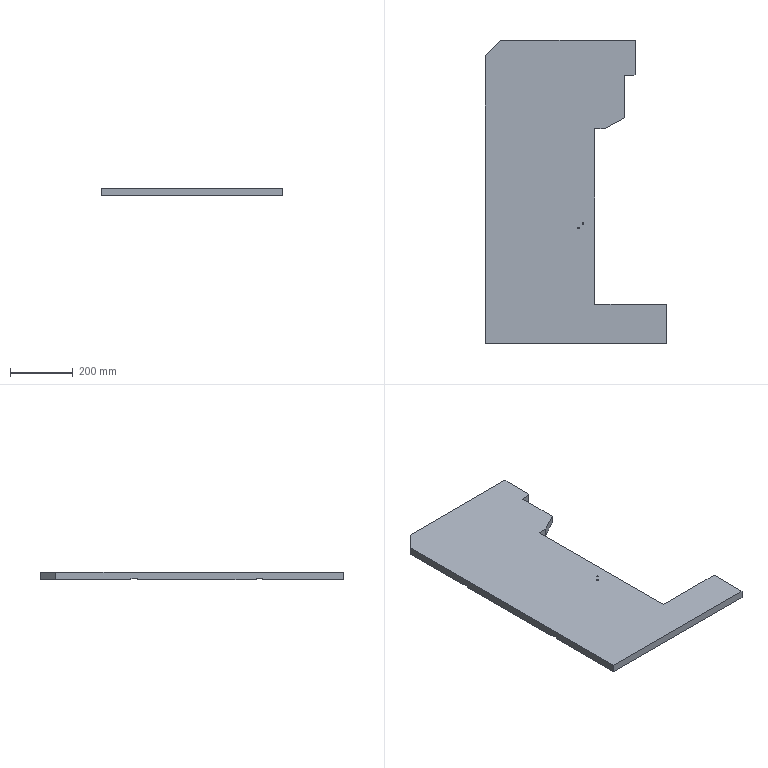Component | SolidWorks | 100-02-1 | 1 solid | 35 faces | box 580 x 970 x 25 mm | volume 9861709 mm3 | plane 23 | cylinder 8 | cone 4 | commonest cylinder face diameters 6.8 x4 5 x4 | material 45
build123d program:
from build123d import *

# Parameters (mm, degrees)
BOSS_EXTRUDE1_DEPTH   = 12.5
CHAMFER1_SIZE         = 5
M6_TAPPED_HOLE1_D     = 5
SKETCH6_W             = 350
SKETCH6_H             = 20
CUT_EXTRUDE1_DEPTH    = 4
LPATTERN1_COUNT       = 2
LPATTERN1_PITCH       = 400
M8_TAPPED_HOLE1_D     = 6.8
M8_TAPPED_HOLE1_DEPTH = 19.75
M8_TAPPED_HOLE1_TIP   = 2.043


with BuildPart() as part:
    # Sketch1 → Boss-Extrude1 (new, symmetric)
    with BuildSketch(Plane.XY):
        Polygon((580, 126), (350, 126), (350, 687), (380, 687), (445, 722), (445, 857), (479, 857), (479, 970), (50, 970), (0, 920), (0, 0), (580, 0), align=None)
    extrude(amount=BOSS_EXTRUDE1_DEPTH, both=True)

    # Chamfer1
    chamfer1_edges = [part.edges().sort_by_distance(p)[0] for p in [
        (479, 857, 0),
    ]]
    chamfer(chamfer1_edges, length=CHAMFER1_SIZE)

    # M6 Tapped Hole1 (through all)
    with Locations(Plane.XY.offset(12.5)):
        with Locations((298, 370), (312.142, 384.142)):
            Hole(M6_TAPPED_HOLE1_D / 2)

    # Sketch6 → Cut-Extrude1 (cut)
    with BuildSketch(Plane(origin=(0, 0, -12.5), x_dir=(-1, 0, 0), z_dir=(0, 0, -1))):
        with Locations((-175, 270)):
            Rectangle(SKETCH6_W, SKETCH6_H)
    cut_extrude1 = extrude(amount=-CUT_EXTRUDE1_DEPTH, mode=Mode.SUBTRACT)

    # LPattern1: Cut-Extrude1 ×2
    with Locations(*[(0, i * LPATTERN1_PITCH, 0) for i in range(1, LPATTERN1_COUNT)]):
        add(cut_extrude1, mode=Mode.SUBTRACT)

    # M8 Tapped Hole1
    with Locations(Plane(origin=(0, 126, 0), x_dir=(1, 0, 0), z_dir=(0, 1, 0))):
        with Locations((552.5, 0), (507.5, 0)):
            Hole(M8_TAPPED_HOLE1_D / 2, depth=M8_TAPPED_HOLE1_DEPTH)
            with Locations((0, 0, -(M8_TAPPED_HOLE1_DEPTH + M8_TAPPED_HOLE1_TIP / 2))):  # 118° drill point
                Cone(0, M8_TAPPED_HOLE1_D / 2, M8_TAPPED_HOLE1_TIP, mode=Mode.SUBTRACT)


solid = part.part

# Placed as in the assembly
solid = solid.moved(Location((-300, 14, 97.5), (0, 0, 0)))
STEP:
#1=COLOUR_RGB('',0.7922,0.8196,0.9333);
#2=FILL_AREA_STYLE_COLOUR('',#1);
#3=FILL_AREA_STYLE('',(#2));
#4=SURFACE_STYLE_FILL_AREA(#3);
#5=SURFACE_SIDE_STYLE('',(#4));
#6=SURFACE_STYLE_USAGE(.BOTH.,#5);
#7=PRESENTATION_STYLE_ASSIGNMENT((#6));
#8=CARTESIAN_POINT('',(9.941,4.734,3.705));
#9=VERTEX_POINT('',#8);
#10=CARTESIAN_POINT('',(9.941,4.734,3.972));
#11=VERTEX_POINT('',#10);
#12=CARTESIAN_POINT('',(9.941,4.734,3.839));
#13=DIRECTION('',(0.,1.,0.));
#14=DIRECTION('',(0.,0.,1.));
#15=AXIS2_PLACEMENT_3D('',#12,#13,#14);
#16=CIRCLE('',#15,0.1339);
#17=EDGE_CURVE('',#9,#11,#16,.T.);
#18=ORIENTED_EDGE('',*,*,#17,.F.);
#19=CARTESIAN_POINT('',(9.941,5.512,3.705));
#20=VERTEX_POINT('',#19);
#21=CARTESIAN_POINT('',(9.941,5.512,3.705));
#22=DIRECTION('',(0.,1.,0.));
#23=VECTOR('',#22,39.37);
#24=LINE('',#21,#23);
#25=EDGE_CURVE('',#9,#20,#24,.T.);
#26=ORIENTED_EDGE('',*,*,#25,.T.);
#27=CARTESIAN_POINT('',(9.941,5.512,3.972));
#28=VERTEX_POINT('',#27);
#29=CARTESIAN_POINT('',(9.941,5.512,3.839));
#30=DIRECTION('',(0.,1.,0.));
#31=DIRECTION('',(0.,0.,1.));
#32=AXIS2_PLACEMENT_3D('',#29,#30,#31);
#33=CIRCLE('',#32,0.1339);
#34=EDGE_CURVE('',#20,#28,#33,.T.);
#35=ORIENTED_EDGE('',*,*,#34,.T.);
#36=CARTESIAN_POINT('',(9.941,5.512,3.972));
#37=DIRECTION('',(0.,1.,0.));
#38=VECTOR('',#37,39.37);
#39=LINE('',#36,#38);
#40=EDGE_CURVE('',#11,#28,#39,.T.);
#41=ORIENTED_EDGE('',*,*,#40,.F.);
#42=EDGE_LOOP('',(#18,#26,#35,#41));
#43=FACE_OUTER_BOUND('',#42,.T.);
#44=CARTESIAN_POINT('',(9.941,5.512,3.839));
#45=DIRECTION('',(0.,1.,0.));
#46=DIRECTION('',(0.,0.,1.));
#47=AXIS2_PLACEMENT_3D('',#44,#45,#46);
#48=CYLINDRICAL_SURFACE('',#47,0.1339);
#49=ADVANCED_FACE('',(#43),#48,.F.);
#50=CARTESIAN_POINT('',(9.941,4.654,3.839));
#51=VERTEX_POINT('',#50);
#52=CARTESIAN_POINT('',(9.941,4.734,3.972));
#53=DIRECTION('',(0.,0.515,0.8572));
#54=VECTOR('',#53,39.37);
#55=LINE('',#52,#54);
#56=EDGE_CURVE('',#51,#11,#55,.T.);
#57=ORIENTED_EDGE('',*,*,#56,.F.);
#58=CARTESIAN_POINT('',(9.941,4.734,3.705));
#59=DIRECTION('',(0.,0.515,-0.8572));
#60=VECTOR('',#59,39.37);
#61=LINE('',#58,#60);
#62=EDGE_CURVE('',#51,#9,#61,.T.);
#63=ORIENTED_EDGE('',*,*,#62,.T.);
#64=ORIENTED_EDGE('',*,*,#17,.T.);
#65=EDGE_LOOP('',(#57,#63,#64));
#66=FACE_OUTER_BOUND('',#65,.T.);
#67=CARTESIAN_POINT('',(9.941,4.734,3.839));
#68=DIRECTION('',(0.,1.,0.));
#69=DIRECTION('',(0.,0.,1.));
#70=AXIS2_PLACEMENT_3D('',#67,#68,#69);
#71=CONICAL_SURFACE('',#70,0.1339,1.03);
#72=ADVANCED_FACE('',(#66),#71,.F.);
#73=CARTESIAN_POINT('',(8.169,4.734,3.705));
#74=VERTEX_POINT('',#73);
#75=CARTESIAN_POINT('',(8.169,4.734,3.972));
#76=VERTEX_POINT('',#75);
#77=CARTESIAN_POINT('',(8.169,4.734,3.839));
#78=DIRECTION('',(0.,1.,0.));
#79=DIRECTION('',(0.,0.,1.));
#80=AXIS2_PLACEMENT_3D('',#77,#78,#79);
#81=CIRCLE('',#80,0.1339);
#82=EDGE_CURVE('',#74,#76,#81,.T.);
#83=ORIENTED_EDGE('',*,*,#82,.F.);
#84=CARTESIAN_POINT('',(8.169,5.512,3.705));
#85=VERTEX_POINT('',#84);
#86=CARTESIAN_POINT('',(8.169,5.512,3.705));
#87=DIRECTION('',(0.,1.,0.));
#88=VECTOR('',#87,39.37);
#89=LINE('',#86,#88);
#90=EDGE_CURVE('',#74,#85,#89,.T.);
#91=ORIENTED_EDGE('',*,*,#90,.T.);
#92=CARTESIAN_POINT('',(8.169,5.512,3.972));
#93=VERTEX_POINT('',#92);
#94=CARTESIAN_POINT('',(8.169,5.512,3.839));
#95=DIRECTION('',(0.,1.,0.));
#96=DIRECTION('',(0.,0.,1.));
#97=AXIS2_PLACEMENT_3D('',#94,#95,#96);
#98=CIRCLE('',#97,0.1339);
#99=EDGE_CURVE('',#85,#93,#98,.T.);
#100=ORIENTED_EDGE('',*,*,#99,.T.);
#101=CARTESIAN_POINT('',(8.169,5.512,3.972));
#102=DIRECTION('',(0.,1.,0.));
#103=VECTOR('',#102,39.37);
#104=LINE('',#101,#103);
#105=EDGE_CURVE('',#76,#93,#104,.T.);
#106=ORIENTED_EDGE('',*,*,#105,.F.);
#107=EDGE_LOOP('',(#83,#91,#100,#106));
#108=FACE_OUTER_BOUND('',#107,.T.);
#109=CARTESIAN_POINT('',(8.169,5.512,3.839));
#110=DIRECTION('',(0.,1.,0.));
#111=DIRECTION('',(0.,0.,1.));
#112=AXIS2_PLACEMENT_3D('',#109,#110,#111);
#113=CYLINDRICAL_SURFACE('',#112,0.1339);
#114=ADVANCED_FACE('',(#108),#113,.F.);
#115=CARTESIAN_POINT('',(8.169,4.654,3.839));
#116=VERTEX_POINT('',#115);
#117=CARTESIAN_POINT('',(8.169,4.734,3.972));
#118=DIRECTION('',(0.,0.515,0.8572));
#119=VECTOR('',#118,39.37);
#120=LINE('',#117,#119);
#121=EDGE_CURVE('',#116,#76,#120,.T.);
#122=ORIENTED_EDGE('',*,*,#121,.F.);
#123=CARTESIAN_POINT('',(8.169,4.734,3.705));
#124=DIRECTION('',(0.,0.515,-0.8572));
#125=VECTOR('',#124,39.37);
#126=LINE('',#123,#125);
#127=EDGE_CURVE('',#116,#74,#126,.T.);
#128=ORIENTED_EDGE('',*,*,#127,.T.);
#129=ORIENTED_EDGE('',*,*,#82,.T.);
#130=EDGE_LOOP('',(#122,#128,#129));
#131=FACE_OUTER_BOUND('',#130,.T.);
#132=CARTESIAN_POINT('',(8.169,4.734,3.839));
#133=DIRECTION('',(0.,1.,0.));
#134=DIRECTION('',(0.,0.,1.));
#135=AXIS2_PLACEMENT_3D('',#132,#133,#134);
#136=CONICAL_SURFACE('',#135,0.1339,1.03);
#137=ADVANCED_FACE('',(#131),#136,.F.);
#138=CARTESIAN_POINT('',(-0.1772,15.118,3.346));
#139=VERTEX_POINT('',#138);
#140=CARTESIAN_POINT('',(0.01969,15.118,3.346));
#141=VERTEX_POINT('',#140);
#142=CARTESIAN_POINT('',(-0.07874,15.118,3.346));
#143=DIRECTION('',(0.,0.,1.));
#144=DIRECTION('',(1.,0.,0.));
#145=AXIS2_PLACEMENT_3D('',#142,#143,#144);
#146=CIRCLE('',#145,0.09843);
#147=EDGE_CURVE('',#139,#141,#146,.T.);
#148=ORIENTED_EDGE('',*,*,#147,.F.);
#149=CARTESIAN_POINT('',(-0.1772,15.118,4.331));
#150=VERTEX_POINT('',#149);
#151=CARTESIAN_POINT('',(-0.1772,15.118,4.331));
#152=DIRECTION('',(0.,0.,1.));
#153=VECTOR('',#152,39.37);
#154=LINE('',#151,#153);
#155=EDGE_CURVE('',#139,#150,#154,.T.);
#156=ORIENTED_EDGE('',*,*,#155,.T.);
#157=CARTESIAN_POINT('',(0.01969,15.118,4.331));
#158=VERTEX_POINT('',#157);
#159=CARTESIAN_POINT('',(-0.07874,15.118,4.331));
#160=DIRECTION('',(0.,0.,1.));
#161=DIRECTION('',(1.,0.,0.));
#162=AXIS2_PLACEMENT_3D('',#159,#160,#161);
#163=CIRCLE('',#162,0.09843);
#164=EDGE_CURVE('',#150,#158,#163,.T.);
#165=ORIENTED_EDGE('',*,*,#164,.T.);
#166=CARTESIAN_POINT('',(0.01969,15.118,4.331));
#167=DIRECTION('',(0.,0.,1.));
#168=VECTOR('',#167,39.37);
#169=LINE('',#166,#168);
#170=EDGE_CURVE('',#141,#158,#169,.T.);
#171=ORIENTED_EDGE('',*,*,#170,.F.);
#172=EDGE_LOOP('',(#148,#156,#165,#171));
#173=FACE_OUTER_BOUND('',#172,.T.);
#174=CARTESIAN_POINT('',(-0.07874,15.118,4.331));
#175=DIRECTION('',(0.,0.,1.));
#176=DIRECTION('',(1.,0.,0.));
#177=AXIS2_PLACEMENT_3D('',#174,#175,#176);
#178=CYLINDRICAL_SURFACE('',#177,0.09843);
#179=ADVANCED_FACE('',(#173),#178,.F.);
#180=CARTESIAN_POINT('',(0.3796,15.675,3.346));
#181=VERTEX_POINT('',#180);
#182=CARTESIAN_POINT('',(0.5765,15.675,3.346));
#183=VERTEX_POINT('',#182);
#184=CARTESIAN_POINT('',(0.478,15.675,3.346));
#185=DIRECTION('',(0.,0.,1.));
#186=DIRECTION('',(1.,0.,0.));
#187=AXIS2_PLACEMENT_3D('',#184,#185,#186);
#188=CIRCLE('',#187,0.09843);
#189=EDGE_CURVE('',#181,#183,#188,.T.);
#190=ORIENTED_EDGE('',*,*,#189,.F.);
#191=CARTESIAN_POINT('',(0.3796,15.675,4.331));
#192=VERTEX_POINT('',#191);
#193=CARTESIAN_POINT('',(0.3796,15.675,4.331));
#194=DIRECTION('',(0.,0.,1.));
#195=VECTOR('',#194,39.37);
#196=LINE('',#193,#195);
#197=EDGE_CURVE('',#181,#192,#196,.T.);
#198=ORIENTED_EDGE('',*,*,#197,.T.);
#199=CARTESIAN_POINT('',(0.5765,15.675,4.331));
#200=VERTEX_POINT('',#199);
#201=CARTESIAN_POINT('',(0.478,15.675,4.331));
#202=DIRECTION('',(0.,0.,1.));
#203=DIRECTION('',(1.,0.,0.));
#204=AXIS2_PLACEMENT_3D('',#201,#202,#203);
#205=CIRCLE('',#204,0.09843);
#206=EDGE_CURVE('',#192,#200,#205,.T.);
#207=ORIENTED_EDGE('',*,*,#206,.T.);
#208=CARTESIAN_POINT('',(0.5765,15.675,4.331));
#209=DIRECTION('',(0.,0.,1.));
#210=VECTOR('',#209,39.37);
#211=LINE('',#208,#210);
#212=EDGE_CURVE('',#183,#200,#211,.T.);
#213=ORIENTED_EDGE('',*,*,#212,.F.);
#214=EDGE_LOOP('',(#190,#198,#207,#213));
#215=FACE_OUTER_BOUND('',#214,.T.);
#216=CARTESIAN_POINT('',(0.478,15.675,4.331));
#217=DIRECTION('',(0.,0.,1.));
#218=DIRECTION('',(1.,0.,0.));
#219=AXIS2_PLACEMENT_3D('',#216,#217,#218);
#220=CYLINDRICAL_SURFACE('',#219,0.09843);
#221=ADVANCED_FACE('',(#215),#220,.F.);
#222=CARTESIAN_POINT('',(1.969,26.535,3.346));
#223=VERTEX_POINT('',#222);
#224=CARTESIAN_POINT('',(-11.811,26.535,3.346));
#225=VERTEX_POINT('',#224);
#226=CARTESIAN_POINT('',(-11.811,26.535,3.346));
#227=DIRECTION('',(-1.,0.,0.));
#228=VECTOR('',#227,39.37);
#229=LINE('',#226,#228);
#230=EDGE_CURVE('',#223,#225,#229,.T.);
#231=ORIENTED_EDGE('',*,*,#230,.F.);
#232=CARTESIAN_POINT('',(1.969,11.575,3.346));
#233=VERTEX_POINT('',#232);
#234=CARTESIAN_POINT('',(1.969,5.512,3.346));
#235=DIRECTION('',(0.,1.,0.));
#236=VECTOR('',#235,39.37);
#237=LINE('',#234,#236);
#238=EDGE_CURVE('',#233,#223,#237,.T.);
#239=ORIENTED_EDGE('',*,*,#238,.F.);
#240=CARTESIAN_POINT('',(-11.811,11.575,3.346));
#241=VERTEX_POINT('',#240);
#242=CARTESIAN_POINT('',(-11.811,11.575,3.346));
#243=DIRECTION('',(1.,-0.,0.));
#244=VECTOR('',#243,39.37);
#245=LINE('',#242,#244);
#246=EDGE_CURVE('',#241,#233,#245,.T.);
#247=ORIENTED_EDGE('',*,*,#246,.F.);
#248=CARTESIAN_POINT('',(-11.811,0.5512,3.346));
#249=DIRECTION('',(-0.,-1.,0.));
#250=VECTOR('',#249,39.37);
#251=LINE('',#248,#250);
#252=EDGE_CURVE('',#225,#241,#251,.T.);
#253=ORIENTED_EDGE('',*,*,#252,.F.);
#254=EDGE_LOOP('',(#231,#239,#247,#253));
#255=FACE_OUTER_BOUND('',#254,.T.);
#256=CARTESIAN_POINT('',(0.478,15.675,3.346));
#257=DIRECTION('',(0.,0.,1.));
#258=DIRECTION('',(1.,0.,0.));
#259=AXIS2_PLACEMENT_3D('',#256,#257,#258);
#260=CIRCLE('',#259,0.09843);
#261=EDGE_CURVE('',#183,#181,#260,.T.);
#262=ORIENTED_EDGE('',*,*,#261,.T.);
#263=ORIENTED_EDGE('',*,*,#189,.T.);
#264=EDGE_LOOP('',(#262,#263));
#265=FACE_BOUND('',#264,.T.);
#266=CARTESIAN_POINT('',(-0.07874,15.118,3.346));
#267=DIRECTION('',(0.,0.,1.));
#268=DIRECTION('',(1.,0.,0.));
#269=AXIS2_PLACEMENT_3D('',#266,#267,#268);
#270=CIRCLE('',#269,0.09843);
#271=EDGE_CURVE('',#141,#139,#270,.T.);
#272=ORIENTED_EDGE('',*,*,#271,.T.);
#273=ORIENTED_EDGE('',*,*,#147,.T.);
#274=EDGE_LOOP('',(#272,#273));
#275=FACE_BOUND('',#274,.T.);
#276=CARTESIAN_POINT('',(-11.811,0.5512,3.346));
#277=DIRECTION('',(0.,0.,-1.));
#278=DIRECTION('',(-1.,0.,0.));
#279=AXIS2_PLACEMENT_3D('',#276,#277,#278);
#280=PLANE('',#279);
#281=ADVANCED_FACE('',(#255,#265,#275),#280,.T.);
#282=CARTESIAN_POINT('',(1.969,10.787,3.346));
#283=VERTEX_POINT('',#282);
#284=CARTESIAN_POINT('',(-11.811,10.787,3.346));
#285=VERTEX_POINT('',#284);
#286=CARTESIAN_POINT('',(-11.811,10.787,3.346));
#287=DIRECTION('',(-1.,0.,0.));
#288=VECTOR('',#287,39.37);
#289=LINE('',#286,#288);
#290=EDGE_CURVE('',#283,#285,#289,.T.);
#291=ORIENTED_EDGE('',*,*,#290,.F.);
#292=CARTESIAN_POINT('',(1.969,5.512,3.346));
#293=VERTEX_POINT('',#292);
#294=CARTESIAN_POINT('',(1.969,5.512,3.346));
#295=DIRECTION('',(0.,1.,0.));
#296=VECTOR('',#295,39.37);
#297=LINE('',#294,#296);
#298=EDGE_CURVE('',#293,#283,#297,.T.);
#299=ORIENTED_EDGE('',*,*,#298,.F.);
#300=CARTESIAN_POINT('',(11.024,5.512,3.346));
#301=VERTEX_POINT('',#300);
#302=CARTESIAN_POINT('',(11.024,5.512,3.346));
#303=DIRECTION('',(-1.,-0.,0.));
#304=VECTOR('',#303,39.37);
#305=LINE('',#302,#304);
#306=EDGE_CURVE('',#301,#293,#305,.T.);
#307=ORIENTED_EDGE('',*,*,#306,.F.);
#308=CARTESIAN_POINT('',(11.024,0.5512,3.346));
#309=VERTEX_POINT('',#308);
#310=CARTESIAN_POINT('',(11.024,0.5512,3.346));
#311=DIRECTION('',(0.,1.,0.));
#312=VECTOR('',#311,39.37);
#313=LINE('',#310,#312);
#314=EDGE_CURVE('',#309,#301,#313,.T.);
#315=ORIENTED_EDGE('',*,*,#314,.F.);
#316=CARTESIAN_POINT('',(-11.811,0.5512,3.346));
#317=VERTEX_POINT('',#316);
#318=CARTESIAN_POINT('',(-11.811,0.5512,3.346));
#319=DIRECTION('',(1.,0.,0.));
#320=VECTOR('',#319,39.37);
#321=LINE('',#318,#320);
#322=EDGE_CURVE('',#317,#309,#321,.T.);
#323=ORIENTED_EDGE('',*,*,#322,.F.);
#324=CARTESIAN_POINT('',(-11.811,0.5512,3.346));
#325=DIRECTION('',(-0.,-1.,0.));
#326=VECTOR('',#325,39.37);
#327=LINE('',#324,#326);
#328=EDGE_CURVE('',#285,#317,#327,.T.);
#329=ORIENTED_EDGE('',*,*,#328,.F.);
#330=EDGE_LOOP('',(#291,#299,#307,#315,#323,#329));
#331=FACE_OUTER_BOUND('',#330,.T.);
#332=CARTESIAN_POINT('',(-11.811,0.5512,3.346));
#333=DIRECTION('',(0.,0.,-1.));
#334=DIRECTION('',(-1.,0.,0.));
#335=AXIS2_PLACEMENT_3D('',#332,#333,#334);
#336=PLANE('',#335);
#337=ADVANCED_FACE('',(#331),#336,.T.);
#338=CARTESIAN_POINT('',(-11.811,27.323,3.346));
#339=VERTEX_POINT('',#338);
#340=CARTESIAN_POINT('',(1.969,27.323,3.346));
#341=VERTEX_POINT('',#340);
#342=CARTESIAN_POINT('',(-11.811,27.323,3.346));
#343=DIRECTION('',(1.,-0.,0.));
#344=VECTOR('',#343,39.37);
#345=LINE('',#342,#344);
#346=EDGE_CURVE('',#339,#341,#345,.T.);
#347=ORIENTED_EDGE('',*,*,#346,.F.);
#348=CARTESIAN_POINT('',(-11.811,36.772,3.346));
#349=VERTEX_POINT('',#348);
#350=CARTESIAN_POINT('',(-11.811,0.5512,3.346));
#351=DIRECTION('',(-0.,-1.,0.));
#352=VECTOR('',#351,39.37);
#353=LINE('',#350,#352);
#354=EDGE_CURVE('',#349,#339,#353,.T.);
#355=ORIENTED_EDGE('',*,*,#354,.F.);
#356=CARTESIAN_POINT('',(-9.843,38.74,3.346));
#357=VERTEX_POINT('',#356);
#358=CARTESIAN_POINT('',(-9.843,38.74,3.346));
#359=DIRECTION('',(-0.7071,-0.7071,0.));
#360=VECTOR('',#359,39.37);
#361=LINE('',#358,#360);
#362=EDGE_CURVE('',#357,#349,#361,.T.);
#363=ORIENTED_EDGE('',*,*,#362,.F.);
#364=CARTESIAN_POINT('',(7.047,38.74,3.346));
#365=VERTEX_POINT('',#364);
#366=CARTESIAN_POINT('',(-9.843,38.74,3.346));
#367=DIRECTION('',(-1.,0.,0.));
#368=VECTOR('',#367,39.37);
#369=LINE('',#366,#368);
#370=EDGE_CURVE('',#365,#357,#369,.T.);
#371=ORIENTED_EDGE('',*,*,#370,.F.);
#372=CARTESIAN_POINT('',(7.047,34.488,3.346));
#373=VERTEX_POINT('',#372);
#374=CARTESIAN_POINT('',(7.047,38.74,3.346));
#375=DIRECTION('',(0.,1.,0.));
#376=VECTOR('',#375,39.37);
#377=LINE('',#374,#376);
#378=EDGE_CURVE('',#373,#365,#377,.T.);
#379=ORIENTED_EDGE('',*,*,#378,.F.);
#380=CARTESIAN_POINT('',(6.85,34.291,3.346));
#381=VERTEX_POINT('',#380);
#382=CARTESIAN_POINT('',(-19.35,8.091,3.346));
#383=DIRECTION('',(-0.7071,-0.7071,0.));
#384=VECTOR('',#383,39.37);
#385=LINE('',#382,#384);
#386=EDGE_CURVE('',#373,#381,#385,.T.);
#387=ORIENTED_EDGE('',*,*,#386,.T.);
#388=CARTESIAN_POINT('',(5.709,34.291,3.346));
#389=VERTEX_POINT('',#388);
#390=CARTESIAN_POINT('',(7.047,34.291,3.346));
#391=DIRECTION('',(1.,0.,0.));
#392=VECTOR('',#391,39.37);
#393=LINE('',#390,#392);
#394=EDGE_CURVE('',#389,#381,#393,.T.);
#395=ORIENTED_EDGE('',*,*,#394,.F.);
#396=CARTESIAN_POINT('',(5.709,28.976,3.346));
#397=VERTEX_POINT('',#396);
#398=CARTESIAN_POINT('',(5.709,34.291,3.346));
#399=DIRECTION('',(0.,1.,0.));
#400=VECTOR('',#399,39.37);
#401=LINE('',#398,#400);
#402=EDGE_CURVE('',#397,#389,#401,.T.);
#403=ORIENTED_EDGE('',*,*,#402,.F.);
#404=CARTESIAN_POINT('',(3.15,27.598,3.346));
#405=VERTEX_POINT('',#404);
#406=CARTESIAN_POINT('',(5.709,28.976,3.346));
#407=DIRECTION('',(0.8805,0.4741,0.));
#408=VECTOR('',#407,39.37);
#409=LINE('',#406,#408);
#410=EDGE_CURVE('',#405,#397,#409,.T.);
#411=ORIENTED_EDGE('',*,*,#410,.F.);
#412=CARTESIAN_POINT('',(1.969,27.598,3.346));
#413=VERTEX_POINT('',#412);
#414=CARTESIAN_POINT('',(1.969,27.598,3.346));
#415=DIRECTION('',(1.,0.,0.));
#416=VECTOR('',#415,39.37);
#417=LINE('',#414,#416);
#418=EDGE_CURVE('',#413,#405,#417,.T.);
#419=ORIENTED_EDGE('',*,*,#418,.F.);
#420=CARTESIAN_POINT('',(1.969,5.512,3.346));
#421=DIRECTION('',(0.,1.,0.));
#422=VECTOR('',#421,39.37);
#423=LINE('',#420,#422);
#424=EDGE_CURVE('',#341,#413,#423,.T.);
#425=ORIENTED_EDGE('',*,*,#424,.F.);
#426=EDGE_LOOP('',(#347,#355,#363,#371,#379,#387,#395,#403,#411,#419,#425));
#427=FACE_OUTER_BOUND('',#426,.T.);
#428=CARTESIAN_POINT('',(-11.811,0.5512,3.346));
#429=DIRECTION('',(0.,0.,-1.));
#430=DIRECTION('',(-1.,0.,0.));
#431=AXIS2_PLACEMENT_3D('',#428,#429,#430);
#432=PLANE('',#431);
#433=ADVANCED_FACE('',(#427),#432,.T.);
#434=CARTESIAN_POINT('',(-11.811,26.535,3.504));
#435=VERTEX_POINT('',#434);
#436=CARTESIAN_POINT('',(-11.811,27.323,3.504));
#437=VERTEX_POINT('',#436);
#438=CARTESIAN_POINT('',(-11.811,26.535,3.504));
#439=DIRECTION('',(0.,1.,0.));
#440=VECTOR('',#439,39.37);
#441=LINE('',#438,#440);
#442=EDGE_CURVE('',#435,#437,#441,.T.);
#443=ORIENTED_EDGE('',*,*,#442,.F.);
#444=CARTESIAN_POINT('',(-11.811,26.535,3.504));
#445=DIRECTION('',(0.,0.,-1.));
#446=VECTOR('',#445,39.37);
#447=LINE('',#444,#446);
#448=EDGE_CURVE('',#435,#225,#447,.T.);
#449=ORIENTED_EDGE('',*,*,#448,.T.);
#450=ORIENTED_EDGE('',*,*,#252,.T.);
#451=CARTESIAN_POINT('',(-11.811,11.575,3.504));
#452=VERTEX_POINT('',#451);
#453=CARTESIAN_POINT('',(-11.811,11.575,3.504));
#454=DIRECTION('',(0.,0.,-1.));
#455=VECTOR('',#454,39.37);
#456=LINE('',#453,#455);
#457=EDGE_CURVE('',#452,#241,#456,.T.);
#458=ORIENTED_EDGE('',*,*,#457,.F.);
#459=CARTESIAN_POINT('',(-11.811,10.787,3.504));
#460=VERTEX_POINT('',#459);
#461=CARTESIAN_POINT('',(-11.811,10.787,3.504));
#462=DIRECTION('',(0.,1.,0.));
#463=VECTOR('',#462,39.37);
#464=LINE('',#461,#463);
#465=EDGE_CURVE('',#460,#452,#464,.T.);
#466=ORIENTED_EDGE('',*,*,#465,.F.);
#467=CARTESIAN_POINT('',(-11.811,10.787,3.504));
#468=DIRECTION('',(0.,0.,-1.));
#469=VECTOR('',#468,39.37);
#470=LINE('',#467,#469);
#471=EDGE_CURVE('',#460,#285,#470,.T.);
#472=ORIENTED_EDGE('',*,*,#471,.T.);
#473=ORIENTED_EDGE('',*,*,#328,.T.);
#474=CARTESIAN_POINT('',(-11.811,0.5512,4.331));
#475=VERTEX_POINT('',#474);
#476=CARTESIAN_POINT('',(-11.811,0.5512,4.331));
#477=DIRECTION('',(0.,0.,-1.));
#478=VECTOR('',#477,39.37);
#479=LINE('',#476,#478);
#480=EDGE_CURVE('',#475,#317,#479,.T.);
#481=ORIENTED_EDGE('',*,*,#480,.F.);
#482=CARTESIAN_POINT('',(-11.811,36.772,4.331));
#483=VERTEX_POINT('',#482);
#484=CARTESIAN_POINT('',(-11.811,0.5512,4.331));
#485=DIRECTION('',(-0.,-1.,0.));
#486=VECTOR('',#485,39.37);
#487=LINE('',#484,#486);
#488=EDGE_CURVE('',#483,#475,#487,.T.);
#489=ORIENTED_EDGE('',*,*,#488,.F.);
#490=CARTESIAN_POINT('',(-11.811,36.772,4.331));
#491=DIRECTION('',(0.,0.,-1.));
#492=VECTOR('',#491,39.37);
#493=LINE('',#490,#492);
#494=EDGE_CURVE('',#483,#349,#493,.T.);
#495=ORIENTED_EDGE('',*,*,#494,.T.);
#496=ORIENTED_EDGE('',*,*,#354,.T.);
#497=CARTESIAN_POINT('',(-11.811,27.323,3.504));
#498=DIRECTION('',(0.,0.,-1.));
#499=VECTOR('',#498,39.37);
#500=LINE('',#497,#499);
#501=EDGE_CURVE('',#437,#339,#500,.T.);
#502=ORIENTED_EDGE('',*,*,#501,.F.);
#503=EDGE_LOOP('',(#443,#449,#450,#458,#466,#472,#473,#481,#489,#495,#496,#502));
#504=FACE_OUTER_BOUND('',#503,.T.);
#505=CARTESIAN_POINT('',(-11.811,0.5512,4.331));
#506=DIRECTION('',(1.,-0.,0.));
#507=DIRECTION('',(0.,1.,0.));
#508=AXIS2_PLACEMENT_3D('',#505,#506,#507);
#509=PLANE('',#508);
#510=ADVANCED_FACE('',(#504),#509,.F.);
#511=ORIENTED_EDGE('',*,*,#322,.T.);
#512=CARTESIAN_POINT('',(11.024,0.5512,4.331));
#513=VERTEX_POINT('',#512);
#514=CARTESIAN_POINT('',(11.024,0.5512,4.331));
#515=DIRECTION('',(0.,0.,-1.));
#516=VECTOR('',#515,39.37);
#517=LINE('',#514,#516);
#518=EDGE_CURVE('',#513,#309,#517,.T.);
#519=ORIENTED_EDGE('',*,*,#518,.F.);
#520=CARTESIAN_POINT('',(-11.811,0.5512,4.331));
#521=DIRECTION('',(1.,0.,0.));
#522=VECTOR('',#521,39.37);
#523=LINE('',#520,#522);
#524=EDGE_CURVE('',#475,#513,#523,.T.);
#525=ORIENTED_EDGE('',*,*,#524,.F.);
#526=ORIENTED_EDGE('',*,*,#480,.T.);
#527=EDGE_LOOP('',(#511,#519,#525,#526));
#528=FACE_OUTER_BOUND('',#527,.T.);
#529=CARTESIAN_POINT('',(-11.811,0.5512,4.331));
#530=DIRECTION('',(0.,1.,0.));
#531=DIRECTION('',(0.,0.,1.));
#532=AXIS2_PLACEMENT_3D('',#529,#530,#531);
#533=PLANE('',#532);
#534=ADVANCED_FACE('',(#528),#533,.F.);
#535=ORIENTED_EDGE('',*,*,#314,.T.);
#536=CARTESIAN_POINT('',(11.024,5.512,4.331));
#537=VERTEX_POINT('',#536);
#538=CARTESIAN_POINT('',(11.024,5.512,4.331));
#539=DIRECTION('',(0.,0.,-1.));
#540=VECTOR('',#539,39.37);
#541=LINE('',#538,#540);
#542=EDGE_CURVE('',#537,#301,#541,.T.);
#543=ORIENTED_EDGE('',*,*,#542,.F.);
#544=CARTESIAN_POINT('',(11.024,0.5512,4.331));
#545=DIRECTION('',(0.,1.,0.));
#546=VECTOR('',#545,39.37);
#547=LINE('',#544,#546);
#548=EDGE_CURVE('',#513,#537,#547,.T.);
#549=ORIENTED_EDGE('',*,*,#548,.F.);
#550=ORIENTED_EDGE('',*,*,#518,.T.);
#551=EDGE_LOOP('',(#535,#543,#549,#550));
#552=FACE_OUTER_BOUND('',#551,.T.);
#553=CARTESIAN_POINT('',(11.024,0.5512,4.331));
#554=DIRECTION('',(-1.,0.,0.));
#555=DIRECTION('',(0.,0.,1.));
#556=AXIS2_PLACEMENT_3D('',#553,#554,#555);
#557=PLANE('',#556);
#558=ADVANCED_FACE('',(#552),#557,.F.);
#559=CARTESIAN_POINT('',(9.941,5.512,3.839));
#560=DIRECTION('',(0.,1.,0.));
#561=DIRECTION('',(0.,0.,1.));
#562=AXIS2_PLACEMENT_3D('',#559,#560,#561);
#563=CIRCLE('',#562,0.1339);
#564=EDGE_CURVE('',#28,#20,#563,.T.);
#565=ORIENTED_EDGE('',*,*,#564,.F.);
#566=ORIENTED_EDGE('',*,*,#34,.F.);
#567=EDGE_LOOP('',(#565,#566));
#568=FACE_BOUND('',#567,.T.);
#569=CARTESIAN_POINT('',(8.169,5.512,3.839));
#570=DIRECTION('',(0.,1.,0.));
#571=DIRECTION('',(0.,0.,1.));
#572=AXIS2_PLACEMENT_3D('',#569,#570,#571);
#573=CIRCLE('',#572,0.1339);
#574=EDGE_CURVE('',#93,#85,#573,.T.);
#575=ORIENTED_EDGE('',*,*,#574,.F.);
#576=ORIENTED_EDGE('',*,*,#99,.F.);
#577=EDGE_LOOP('',(#575,#576));
#578=FACE_BOUND('',#577,.T.);
#579=ORIENTED_EDGE('',*,*,#306,.T.);
#580=CARTESIAN_POINT('',(1.969,5.512,4.331));
#581=VERTEX_POINT('',#580);
#582=CARTESIAN_POINT('',(1.969,5.512,4.331));
#583=DIRECTION('',(0.,0.,-1.));
#584=VECTOR('',#583,39.37);
#585=LINE('',#582,#584);
#586=EDGE_CURVE('',#581,#293,#585,.T.);
#587=ORIENTED_EDGE('',*,*,#586,.F.);
#588=CARTESIAN_POINT('',(11.024,5.512,4.331));
#589=DIRECTION('',(-1.,-0.,0.));
#590=VECTOR('',#589,39.37);
#591=LINE('',#588,#590);
#592=EDGE_CURVE('',#537,#581,#591,.T.);
#593=ORIENTED_EDGE('',*,*,#592,.F.);
#594=ORIENTED_EDGE('',*,*,#542,.T.);
#595=EDGE_LOOP('',(#579,#587,#593,#594));
#596=FACE_OUTER_BOUND('',#595,.T.);
#597=CARTESIAN_POINT('',(11.024,5.512,4.331));
#598=DIRECTION('',(0.,-1.,0.));
#599=DIRECTION('',(1.,0.,0.));
#600=AXIS2_PLACEMENT_3D('',#597,#598,#599);
#601=PLANE('',#600);
#602=ADVANCED_FACE('',(#568,#578,#596),#601,.F.);
#603=ORIENTED_EDGE('',*,*,#238,.T.);
#604=CARTESIAN_POINT('',(1.969,26.535,3.504));
#605=VERTEX_POINT('',#604);
#606=CARTESIAN_POINT('',(1.969,26.535,3.504));
#607=DIRECTION('',(0.,0.,-1.));
#608=VECTOR('',#607,39.37);
#609=LINE('',#606,#608);
#610=EDGE_CURVE('',#605,#223,#609,.T.);
#611=ORIENTED_EDGE('',*,*,#610,.F.);
#612=CARTESIAN_POINT('',(1.969,27.323,3.504));
#613=VERTEX_POINT('',#612);
#614=CARTESIAN_POINT('',(1.969,26.535,3.504));
#615=DIRECTION('',(0.,-1.,0.));
#616=VECTOR('',#615,39.37);
#617=LINE('',#614,#616);
#618=EDGE_CURVE('',#613,#605,#617,.T.);
#619=ORIENTED_EDGE('',*,*,#618,.F.);
#620=CARTESIAN_POINT('',(1.969,27.323,3.504));
#621=DIRECTION('',(0.,0.,-1.));
#622=VECTOR('',#621,39.37);
#623=LINE('',#620,#622);
#624=EDGE_CURVE('',#613,#341,#623,.T.);
#625=ORIENTED_EDGE('',*,*,#624,.T.);
#626=ORIENTED_EDGE('',*,*,#424,.T.);
#627=CARTESIAN_POINT('',(1.969,27.598,4.331));
#628=VERTEX_POINT('',#627);
#629=CARTESIAN_POINT('',(1.969,27.598,4.331));
#630=DIRECTION('',(0.,0.,-1.));
#631=VECTOR('',#630,39.37);
#632=LINE('',#629,#631);
#633=EDGE_CURVE('',#628,#413,#632,.T.);
#634=ORIENTED_EDGE('',*,*,#633,.F.);
#635=CARTESIAN_POINT('',(1.969,5.512,4.331));
#636=DIRECTION('',(0.,1.,0.));
#637=VECTOR('',#636,39.37);
#638=LINE('',#635,#637);
#639=EDGE_CURVE('',#581,#628,#638,.T.);
#640=ORIENTED_EDGE('',*,*,#639,.F.);
#641=ORIENTED_EDGE('',*,*,#586,.T.);
#642=ORIENTED_EDGE('',*,*,#298,.T.);
#643=CARTESIAN_POINT('',(1.969,10.787,3.504));
#644=VERTEX_POINT('',#643);
#645=CARTESIAN_POINT('',(1.969,10.787,3.504));
#646=DIRECTION('',(0.,0.,-1.));
#647=VECTOR('',#646,39.37);
#648=LINE('',#645,#647);
#649=EDGE_CURVE('',#644,#283,#648,.T.);
#650=ORIENTED_EDGE('',*,*,#649,.F.);
#651=CARTESIAN_POINT('',(1.969,11.575,3.504));
#652=VERTEX_POINT('',#651);
#653=CARTESIAN_POINT('',(1.969,10.787,3.504));
#654=DIRECTION('',(0.,-1.,0.));
#655=VECTOR('',#654,39.37);
#656=LINE('',#653,#655);
#657=EDGE_CURVE('',#652,#644,#656,.T.);
#658=ORIENTED_EDGE('',*,*,#657,.F.);
#659=CARTESIAN_POINT('',(1.969,11.575,3.504));
#660=DIRECTION('',(0.,0.,-1.));
#661=VECTOR('',#660,39.37);
#662=LINE('',#659,#661);
#663=EDGE_CURVE('',#652,#233,#662,.T.);
#664=ORIENTED_EDGE('',*,*,#663,.T.);
#665=EDGE_LOOP('',(#603,#611,#619,#625,#626,#634,#640,#641,#642,#650,#658,#664));
#666=FACE_OUTER_BOUND('',#665,.T.);
#667=CARTESIAN_POINT('',(1.969,5.512,4.331));
#668=DIRECTION('',(-1.,0.,0.));
#669=DIRECTION('',(0.,0.,1.));
#670=AXIS2_PLACEMENT_3D('',#667,#668,#669);
#671=PLANE('',#670);
#672=ADVANCED_FACE('',(#666),#671,.F.);
#673=ORIENTED_EDGE('',*,*,#418,.T.);
#674=CARTESIAN_POINT('',(3.15,27.598,4.331));
#675=VERTEX_POINT('',#674);
#676=CARTESIAN_POINT('',(3.15,27.598,4.331));
#677=DIRECTION('',(0.,0.,-1.));
#678=VECTOR('',#677,39.37);
#679=LINE('',#676,#678);
#680=EDGE_CURVE('',#675,#405,#679,.T.);
#681=ORIENTED_EDGE('',*,*,#680,.F.);
#682=CARTESIAN_POINT('',(1.969,27.598,4.331));
#683=DIRECTION('',(1.,0.,0.));
#684=VECTOR('',#683,39.37);
#685=LINE('',#682,#684);
#686=EDGE_CURVE('',#628,#675,#685,.T.);
#687=ORIENTED_EDGE('',*,*,#686,.F.);
#688=ORIENTED_EDGE('',*,*,#633,.T.);
#689=EDGE_LOOP('',(#673,#681,#687,#688));
#690=FACE_OUTER_BOUND('',#689,.T.);
#691=CARTESIAN_POINT('',(1.969,27.598,4.331));
#692=DIRECTION('',(-0.,1.,0.));
#693=DIRECTION('',(-1.,-0.,0.));
#694=AXIS2_PLACEMENT_3D('',#691,#692,#693);
#695=PLANE('',#694);
#696=ADVANCED_FACE('',(#690),#695,.F.);
#697=ORIENTED_EDGE('',*,*,#410,.T.);
#698=CARTESIAN_POINT('',(5.709,28.976,4.331));
#699=VERTEX_POINT('',#698);
#700=CARTESIAN_POINT('',(5.709,28.976,4.331));
#701=DIRECTION('',(0.,0.,-1.));
#702=VECTOR('',#701,39.37);
#703=LINE('',#700,#702);
#704=EDGE_CURVE('',#699,#397,#703,.T.);
#705=ORIENTED_EDGE('',*,*,#704,.F.);
#706=CARTESIAN_POINT('',(5.709,28.976,4.331));
#707=DIRECTION('',(0.8805,0.4741,0.));
#708=VECTOR('',#707,39.37);
#709=LINE('',#706,#708);
#710=EDGE_CURVE('',#675,#699,#709,.T.);
#711=ORIENTED_EDGE('',*,*,#710,.F.);
#712=ORIENTED_EDGE('',*,*,#680,.T.);
#713=EDGE_LOOP('',(#697,#705,#711,#712));
#714=FACE_OUTER_BOUND('',#713,.T.);
#715=CARTESIAN_POINT('',(5.709,28.976,4.331));
#716=DIRECTION('',(-0.4741,0.8805,0.));
#717=DIRECTION('',(-0.8805,-0.4741,0.));
#718=AXIS2_PLACEMENT_3D('',#715,#716,#717);
#719=PLANE('',#718);
#720=ADVANCED_FACE('',(#714),#719,.F.);
#721=ORIENTED_EDGE('',*,*,#402,.T.);
#722=CARTESIAN_POINT('',(5.709,34.291,4.331));
#723=VERTEX_POINT('',#722);
#724=CARTESIAN_POINT('',(5.709,34.291,4.331));
#725=DIRECTION('',(0.,0.,-1.));
#726=VECTOR('',#725,39.37);
#727=LINE('',#724,#726);
#728=EDGE_CURVE('',#723,#389,#727,.T.);
#729=ORIENTED_EDGE('',*,*,#728,.F.);
#730=CARTESIAN_POINT('',(5.709,34.291,4.331));
#731=DIRECTION('',(0.,1.,0.));
#732=VECTOR('',#731,39.37);
#733=LINE('',#730,#732);
#734=EDGE_CURVE('',#699,#723,#733,.T.);
#735=ORIENTED_EDGE('',*,*,#734,.F.);
#736=ORIENTED_EDGE('',*,*,#704,.T.);
#737=EDGE_LOOP('',(#721,#729,#735,#736));
#738=FACE_OUTER_BOUND('',#737,.T.);
#739=CARTESIAN_POINT('',(5.709,34.291,4.331));
#740=DIRECTION('',(-1.,0.,0.));
#741=DIRECTION('',(-0.,-1.,0.));
#742=AXIS2_PLACEMENT_3D('',#739,#740,#741);
#743=PLANE('',#742);
#744=ADVANCED_FACE('',(#738),#743,.F.);
#745=ORIENTED_EDGE('',*,*,#394,.T.);
#746=CARTESIAN_POINT('',(6.85,34.291,4.331));
#747=VERTEX_POINT('',#746);
#748=CARTESIAN_POINT('',(6.85,34.291,4.331));
#749=DIRECTION('',(0.,0.,1.));
#750=VECTOR('',#749,39.37);
#751=LINE('',#748,#750);
#752=EDGE_CURVE('',#381,#747,#751,.T.);
#753=ORIENTED_EDGE('',*,*,#752,.T.);
#754=CARTESIAN_POINT('',(7.047,34.291,4.331));
#755=DIRECTION('',(1.,0.,0.));
#756=VECTOR('',#755,39.37);
#757=LINE('',#754,#756);
#758=EDGE_CURVE('',#723,#747,#757,.T.);
#759=ORIENTED_EDGE('',*,*,#758,.F.);
#760=ORIENTED_EDGE('',*,*,#728,.T.);
#761=EDGE_LOOP('',(#745,#753,#759,#760));
#762=FACE_OUTER_BOUND('',#761,.T.);
#763=CARTESIAN_POINT('',(7.047,34.291,4.331));
#764=DIRECTION('',(0.,1.,0.));
#765=DIRECTION('',(0.,0.,1.));
#766=AXIS2_PLACEMENT_3D('',#763,#764,#765);
#767=PLANE('',#766);
#768=ADVANCED_FACE('',(#762),#767,.F.);
#769=CARTESIAN_POINT('',(7.047,34.488,4.331));
#770=VERTEX_POINT('',#769);
#771=CARTESIAN_POINT('',(7.047,38.74,4.331));
#772=VERTEX_POINT('',#771);
#773=CARTESIAN_POINT('',(7.047,38.74,4.331));
#774=DIRECTION('',(0.,1.,0.));
#775=VECTOR('',#774,39.37);
#776=LINE('',#773,#775);
#777=EDGE_CURVE('',#770,#772,#776,.T.);
#778=ORIENTED_EDGE('',*,*,#777,.F.);
#779=CARTESIAN_POINT('',(7.047,34.488,4.331));
#780=DIRECTION('',(0.,0.,-1.));
#781=VECTOR('',#780,39.37);
#782=LINE('',#779,#781);
#783=EDGE_CURVE('',#770,#373,#782,.T.);
#784=ORIENTED_EDGE('',*,*,#783,.T.);
#785=ORIENTED_EDGE('',*,*,#378,.T.);
#786=CARTESIAN_POINT('',(7.047,38.74,4.331));
#787=DIRECTION('',(0.,0.,-1.));
#788=VECTOR('',#787,39.37);
#789=LINE('',#786,#788);
#790=EDGE_CURVE('',#772,#365,#789,.T.);
#791=ORIENTED_EDGE('',*,*,#790,.F.);
#792=EDGE_LOOP('',(#778,#784,#785,#791));
#793=FACE_OUTER_BOUND('',#792,.T.);
#794=CARTESIAN_POINT('',(7.047,38.74,4.331));
#795=DIRECTION('',(-1.,0.,0.));
#796=DIRECTION('',(0.,0.,1.));
#797=AXIS2_PLACEMENT_3D('',#794,#795,#796);
#798=PLANE('',#797);
#799=ADVANCED_FACE('',(#793),#798,.F.);
#800=ORIENTED_EDGE('',*,*,#370,.T.);
#801=CARTESIAN_POINT('',(-9.843,38.74,4.331));
#802=VERTEX_POINT('',#801);
#803=CARTESIAN_POINT('',(-9.843,38.74,4.331));
#804=DIRECTION('',(0.,0.,-1.));
#805=VECTOR('',#804,39.37);
#806=LINE('',#803,#805);
#807=EDGE_CURVE('',#802,#357,#806,.T.);
#808=ORIENTED_EDGE('',*,*,#807,.F.);
#809=CARTESIAN_POINT('',(-9.843,38.74,4.331));
#810=DIRECTION('',(-1.,0.,0.));
#811=VECTOR('',#810,39.37);
#812=LINE('',#809,#811);
#813=EDGE_CURVE('',#772,#802,#812,.T.);
#814=ORIENTED_EDGE('',*,*,#813,.F.);
#815=ORIENTED_EDGE('',*,*,#790,.T.);
#816=EDGE_LOOP('',(#800,#808,#814,#815));
#817=FACE_OUTER_BOUND('',#816,.T.);
#818=CARTESIAN_POINT('',(-9.843,38.74,4.331));
#819=DIRECTION('',(0.,-1.,0.));
#820=DIRECTION('',(0.,0.,-1.));
#821=AXIS2_PLACEMENT_3D('',#818,#819,#820);
#822=PLANE('',#821);
#823=ADVANCED_FACE('',(#817),#822,.F.);
#824=ORIENTED_EDGE('',*,*,#362,.T.);
#825=ORIENTED_EDGE('',*,*,#494,.F.);
#826=CARTESIAN_POINT('',(-9.843,38.74,4.331));
#827=DIRECTION('',(-0.7071,-0.7071,0.));
#828=VECTOR('',#827,39.37);
#829=LINE('',#826,#828);
#830=EDGE_CURVE('',#802,#483,#829,.T.);
#831=ORIENTED_EDGE('',*,*,#830,.F.);
#832=ORIENTED_EDGE('',*,*,#807,.T.);
#833=EDGE_LOOP('',(#824,#825,#831,#832));
#834=FACE_OUTER_BOUND('',#833,.T.);
#835=CARTESIAN_POINT('',(-9.843,38.74,4.331));
#836=DIRECTION('',(0.7071,-0.7071,0.));
#837=DIRECTION('',(0.7071,0.7071,0.));
#838=AXIS2_PLACEMENT_3D('',#835,#836,#837);
#839=PLANE('',#838);
#840=ADVANCED_FACE('',(#834),#839,.F.);
#841=CARTESIAN_POINT('',(-0.07874,15.118,4.331));
#842=DIRECTION('',(0.,0.,1.));
#843=DIRECTION('',(1.,0.,0.));
#844=AXIS2_PLACEMENT_3D('',#841,#842,#843);
#845=CIRCLE('',#844,0.09843);
#846=EDGE_CURVE('',#158,#150,#845,.T.);
#847=ORIENTED_EDGE('',*,*,#846,.F.);
#848=ORIENTED_EDGE('',*,*,#164,.F.);
#849=EDGE_LOOP('',(#847,#848));
#850=FACE_BOUND('',#849,.T.);
#851=CARTESIAN_POINT('',(0.478,15.675,4.331));
#852=DIRECTION('',(0.,0.,1.));
#853=DIRECTION('',(1.,0.,0.));
#854=AXIS2_PLACEMENT_3D('',#851,#852,#853);
#855=CIRCLE('',#854,0.09843);
#856=EDGE_CURVE('',#200,#192,#855,.T.);
#857=ORIENTED_EDGE('',*,*,#856,.F.);
#858=ORIENTED_EDGE('',*,*,#206,.F.);
#859=EDGE_LOOP('',(#857,#858));
#860=FACE_BOUND('',#859,.T.);
#861=ORIENTED_EDGE('',*,*,#758,.T.);
#862=CARTESIAN_POINT('',(7.047,34.488,4.331));
#863=DIRECTION('',(0.7071,0.7071,0.));
#864=VECTOR('',#863,39.37);
#865=LINE('',#862,#864);
#866=EDGE_CURVE('',#747,#770,#865,.T.);
#867=ORIENTED_EDGE('',*,*,#866,.T.);
#868=ORIENTED_EDGE('',*,*,#777,.T.);
#869=ORIENTED_EDGE('',*,*,#813,.T.);
#870=ORIENTED_EDGE('',*,*,#830,.T.);
#871=ORIENTED_EDGE('',*,*,#488,.T.);
#872=ORIENTED_EDGE('',*,*,#524,.T.);
#873=ORIENTED_EDGE('',*,*,#548,.T.);
#874=ORIENTED_EDGE('',*,*,#592,.T.);
#875=ORIENTED_EDGE('',*,*,#639,.T.);
#876=ORIENTED_EDGE('',*,*,#686,.T.);
#877=ORIENTED_EDGE('',*,*,#710,.T.);
#878=ORIENTED_EDGE('',*,*,#734,.T.);
#879=EDGE_LOOP('',(#861,#867,#868,#869,#870,#871,#872,#873,#874,#875,#876,#877,#878));
#880=FACE_OUTER_BOUND('',#879,.T.);
#881=CARTESIAN_POINT('',(-11.811,0.5512,4.331));
#882=DIRECTION('',(0.,0.,-1.));
#883=DIRECTION('',(-1.,0.,0.));
#884=AXIS2_PLACEMENT_3D('',#881,#882,#883);
#885=PLANE('',#884);
#886=ADVANCED_FACE('',(#850,#860,#880),#885,.F.);
#887=ORIENTED_EDGE('',*,*,#866,.F.);
#888=ORIENTED_EDGE('',*,*,#752,.F.);
#889=ORIENTED_EDGE('',*,*,#386,.F.);
#890=ORIENTED_EDGE('',*,*,#783,.F.);
#891=EDGE_LOOP('',(#887,#888,#889,#890));
#892=FACE_OUTER_BOUND('',#891,.T.);
#893=CARTESIAN_POINT('',(7.047,34.488,4.331));
#894=DIRECTION('',(-0.7071,0.7071,0.));
#895=DIRECTION('',(0.,0.,-1.));
#896=AXIS2_PLACEMENT_3D('',#893,#894,#895);
#897=PLANE('',#896);
#898=ADVANCED_FACE('',(#892),#897,.F.);
#899=ORIENTED_EDGE('',*,*,#197,.F.);
#900=ORIENTED_EDGE('',*,*,#261,.F.);
#901=ORIENTED_EDGE('',*,*,#212,.T.);
#902=ORIENTED_EDGE('',*,*,#856,.T.);
#903=EDGE_LOOP('',(#899,#900,#901,#902));
#904=FACE_OUTER_BOUND('',#903,.T.);
#905=CARTESIAN_POINT('',(0.478,15.675,4.331));
#906=DIRECTION('',(0.,0.,1.));
#907=DIRECTION('',(1.,0.,0.));
#908=AXIS2_PLACEMENT_3D('',#905,#906,#907);
#909=CYLINDRICAL_SURFACE('',#908,0.09843);
#910=ADVANCED_FACE('',(#904),#909,.F.);
#911=ORIENTED_EDGE('',*,*,#155,.F.);
#912=ORIENTED_EDGE('',*,*,#271,.F.);
#913=ORIENTED_EDGE('',*,*,#170,.T.);
#914=ORIENTED_EDGE('',*,*,#846,.T.);
#915=EDGE_LOOP('',(#911,#912,#913,#914));
#916=FACE_OUTER_BOUND('',#915,.T.);
#917=CARTESIAN_POINT('',(-0.07874,15.118,4.331));
#918=DIRECTION('',(0.,0.,1.));
#919=DIRECTION('',(1.,0.,0.));
#920=AXIS2_PLACEMENT_3D('',#917,#918,#919);
#921=CYLINDRICAL_SURFACE('',#920,0.09843);
#922=ADVANCED_FACE('',(#916),#921,.F.);
#923=ORIENTED_EDGE('',*,*,#290,.T.);
#924=ORIENTED_EDGE('',*,*,#471,.F.);
#925=CARTESIAN_POINT('',(-11.811,10.787,3.504));
#926=DIRECTION('',(-1.,0.,0.));
#927=VECTOR('',#926,39.37);
#928=LINE('',#925,#927);
#929=EDGE_CURVE('',#644,#460,#928,.T.);
#930=ORIENTED_EDGE('',*,*,#929,.F.);
#931=ORIENTED_EDGE('',*,*,#649,.T.);
#932=EDGE_LOOP('',(#923,#924,#930,#931));
#933=FACE_OUTER_BOUND('',#932,.T.);
#934=CARTESIAN_POINT('',(-11.811,10.787,3.504));
#935=DIRECTION('',(-0.,-1.,0.));
#936=DIRECTION('',(1.,-0.,0.));
#937=AXIS2_PLACEMENT_3D('',#934,#935,#936);
#938=PLANE('',#937);
#939=ADVANCED_FACE('',(#933),#938,.F.);
#940=ORIENTED_EDGE('',*,*,#246,.T.);
#941=ORIENTED_EDGE('',*,*,#663,.F.);
#942=CARTESIAN_POINT('',(-11.811,11.575,3.504));
#943=DIRECTION('',(1.,-0.,0.));
#944=VECTOR('',#943,39.37);
#945=LINE('',#942,#944);
#946=EDGE_CURVE('',#452,#652,#945,.T.);
#947=ORIENTED_EDGE('',*,*,#946,.F.);
#948=ORIENTED_EDGE('',*,*,#457,.T.);
#949=EDGE_LOOP('',(#940,#941,#947,#948));
#950=FACE_OUTER_BOUND('',#949,.T.);
#951=CARTESIAN_POINT('',(-11.811,11.575,3.504));
#952=DIRECTION('',(0.,1.,0.));
#953=DIRECTION('',(-1.,0.,0.));
#954=AXIS2_PLACEMENT_3D('',#951,#952,#953);
#955=PLANE('',#954);
#956=ADVANCED_FACE('',(#950),#955,.F.);
#957=ORIENTED_EDGE('',*,*,#465,.T.);
#958=ORIENTED_EDGE('',*,*,#946,.T.);
#959=ORIENTED_EDGE('',*,*,#657,.T.);
#960=ORIENTED_EDGE('',*,*,#929,.T.);
#961=EDGE_LOOP('',(#957,#958,#959,#960));
#962=FACE_OUTER_BOUND('',#961,.T.);
#963=CARTESIAN_POINT('',(-11.811,0.5512,3.504));
#964=DIRECTION('',(0.,0.,-1.));
#965=DIRECTION('',(-1.,0.,0.));
#966=AXIS2_PLACEMENT_3D('',#963,#964,#965);
#967=PLANE('',#966);
#968=ADVANCED_FACE('',(#962),#967,.T.);
#969=ORIENTED_EDGE('',*,*,#230,.T.);
#970=ORIENTED_EDGE('',*,*,#448,.F.);
#971=CARTESIAN_POINT('',(-11.811,26.535,3.504));
#972=DIRECTION('',(-1.,0.,0.));
#973=VECTOR('',#972,39.37);
#974=LINE('',#971,#973);
#975=EDGE_CURVE('',#605,#435,#974,.T.);
#976=ORIENTED_EDGE('',*,*,#975,.F.);
#977=ORIENTED_EDGE('',*,*,#610,.T.);
#978=EDGE_LOOP('',(#969,#970,#976,#977));
#979=FACE_OUTER_BOUND('',#978,.T.);
#980=CARTESIAN_POINT('',(-11.811,26.535,3.504));
#981=DIRECTION('',(-0.,-1.,0.));
#982=DIRECTION('',(1.,-0.,0.));
#983=AXIS2_PLACEMENT_3D('',#980,#981,#982);
#984=PLANE('',#983);
#985=ADVANCED_FACE('',(#979),#984,.F.);
#986=ORIENTED_EDGE('',*,*,#346,.T.);
#987=ORIENTED_EDGE('',*,*,#624,.F.);
#988=CARTESIAN_POINT('',(-11.811,27.323,3.504));
#989=DIRECTION('',(1.,-0.,0.));
#990=VECTOR('',#989,39.37);
#991=LINE('',#988,#990);
#992=EDGE_CURVE('',#437,#613,#991,.T.);
#993=ORIENTED_EDGE('',*,*,#992,.F.);
#994=ORIENTED_EDGE('',*,*,#501,.T.);
#995=EDGE_LOOP('',(#986,#987,#993,#994));
#996=FACE_OUTER_BOUND('',#995,.T.);
#997=CARTESIAN_POINT('',(-11.811,27.323,3.504));
#998=DIRECTION('',(0.,1.,0.));
#999=DIRECTION('',(-1.,0.,0.));
#1000=AXIS2_PLACEMENT_3D('',#997,#998,#999);
#1001=PLANE('',#1000);
#1002=ADVANCED_FACE('',(#996),#1001,.F.);
#1003=ORIENTED_EDGE('',*,*,#442,.T.);
#1004=ORIENTED_EDGE('',*,*,#992,.T.);
#1005=ORIENTED_EDGE('',*,*,#618,.T.);
#1006=ORIENTED_EDGE('',*,*,#975,.T.);
#1007=EDGE_LOOP('',(#1003,#1004,#1005,#1006));
#1008=FACE_OUTER_BOUND('',#1007,.T.);
#1009=CARTESIAN_POINT('',(-11.811,16.299,3.504));
#1010=DIRECTION('',(0.,0.,-1.));
#1011=DIRECTION('',(-1.,0.,0.));
#1012=AXIS2_PLACEMENT_3D('',#1009,#1010,#1011);
#1013=PLANE('',#1012);
#1014=ADVANCED_FACE('',(#1008),#1013,.T.);
#1015=ORIENTED_EDGE('',*,*,#127,.F.);
#1016=ORIENTED_EDGE('',*,*,#121,.T.);
#1017=CARTESIAN_POINT('',(8.169,4.734,3.839));
#1018=DIRECTION('',(0.,1.,0.));
#1019=DIRECTION('',(0.,0.,1.));
#1020=AXIS2_PLACEMENT_3D('',#1017,#1018,#1019);
#1021=CIRCLE('',#1020,0.1339);
#1022=EDGE_CURVE('',#76,#74,#1021,.T.);
#1023=ORIENTED_EDGE('',*,*,#1022,.T.);
#1024=EDGE_LOOP('',(#1015,#1016,#1023));
#1025=FACE_OUTER_BOUND('',#1024,.T.);
#1026=CARTESIAN_POINT('',(8.169,4.734,3.839));
#1027=DIRECTION('',(0.,1.,0.));
#1028=DIRECTION('',(0.,0.,1.));
#1029=AXIS2_PLACEMENT_3D('',#1026,#1027,#1028);
#1030=CONICAL_SURFACE('',#1029,0.1339,1.03);
#1031=ADVANCED_FACE('',(#1025),#1030,.F.);
#1032=ORIENTED_EDGE('',*,*,#90,.F.);
#1033=ORIENTED_EDGE('',*,*,#1022,.F.);
#1034=ORIENTED_EDGE('',*,*,#105,.T.);
#1035=ORIENTED_EDGE('',*,*,#574,.T.);
#1036=EDGE_LOOP('',(#1032,#1033,#1034,#1035));
#1037=FACE_OUTER_BOUND('',#1036,.T.);
#1038=CARTESIAN_POINT('',(8.169,5.512,3.839));
#1039=DIRECTION('',(0.,1.,0.));
#1040=DIRECTION('',(0.,0.,1.));
#1041=AXIS2_PLACEMENT_3D('',#1038,#1039,#1040);
#1042=CYLINDRICAL_SURFACE('',#1041,0.1339);
#1043=ADVANCED_FACE('',(#1037),#1042,.F.);
#1044=ORIENTED_EDGE('',*,*,#62,.F.);
#1045=ORIENTED_EDGE('',*,*,#56,.T.);
#1046=CARTESIAN_POINT('',(9.941,4.734,3.839));
#1047=DIRECTION('',(0.,1.,0.));
#1048=DIRECTION('',(0.,0.,1.));
#1049=AXIS2_PLACEMENT_3D('',#1046,#1047,#1048);
#1050=CIRCLE('',#1049,0.1339);
#1051=EDGE_CURVE('',#11,#9,#1050,.T.);
#1052=ORIENTED_EDGE('',*,*,#1051,.T.);
#1053=EDGE_LOOP('',(#1044,#1045,#1052));
#1054=FACE_OUTER_BOUND('',#1053,.T.);
#1055=CARTESIAN_POINT('',(9.941,4.734,3.839));
#1056=DIRECTION('',(0.,1.,0.));
#1057=DIRECTION('',(0.,0.,1.));
#1058=AXIS2_PLACEMENT_3D('',#1055,#1056,#1057);
#1059=CONICAL_SURFACE('',#1058,0.1339,1.03);
#1060=ADVANCED_FACE('',(#1054),#1059,.F.);
#1061=ORIENTED_EDGE('',*,*,#25,.F.);
#1062=ORIENTED_EDGE('',*,*,#1051,.F.);
#1063=ORIENTED_EDGE('',*,*,#40,.T.);
#1064=ORIENTED_EDGE('',*,*,#564,.T.);
#1065=EDGE_LOOP('',(#1061,#1062,#1063,#1064));
#1066=FACE_OUTER_BOUND('',#1065,.T.);
#1067=CARTESIAN_POINT('',(9.941,5.512,3.839));
#1068=DIRECTION('',(0.,1.,0.));
#1069=DIRECTION('',(0.,0.,1.));
#1070=AXIS2_PLACEMENT_3D('',#1067,#1068,#1069);
#1071=CYLINDRICAL_SURFACE('',#1070,0.1339);
#1072=ADVANCED_FACE('',(#1066),#1071,.F.);
#1073=CLOSED_SHELL('',(#49,#72,#114,#137,#179,#221,#281,#337,#433,#510,#534,#558,#602,#672,#696,#720,#744,#768,#799,#823,#840,#886,#898,#910,#922,#939,#956,#968,#985,#1002,#1014,#1031,#1043,#1060,#1072));
#1074=MANIFOLD_SOLID_BREP('',#1073);
#1075=STYLED_ITEM('',(#7),#1074);
#1076=PRESENTATION_LAYER_ASSIGNMENT('','',(#1075));
#1077=CARTESIAN_POINT('',(0.,0.,0.));
#1078=DIRECTION('',(0.,0.,1.));
#1079=DIRECTION('',(1.,0.,0.));
#1080=AXIS2_PLACEMENT_3D('',#1077,#1078,#1079);
#1081=(LENGTH_UNIT()NAMED_UNIT(*)SI_UNIT($,.METRE.));
#1082=LENGTH_MEASURE_WITH_UNIT(LENGTH_MEASURE(0.0254),#1081);
#1083=DIMENSIONAL_EXPONENTS(1.,0.,0.,0.,0.,0.,0.);
#1084=(CONVERSION_BASED_UNIT('',#1082)LENGTH_UNIT()NAMED_UNIT(#1083));
#1085=UNCERTAINTY_MEASURE_WITH_UNIT(LENGTH_MEASURE(0.00001),#1084,'','');
#1086=(NAMED_UNIT(*)PLANE_ANGLE_UNIT()SI_UNIT($,.RADIAN.));
#1087=(NAMED_UNIT(*)SI_UNIT($,.STERADIAN.)SOLID_ANGLE_UNIT());
#1088=(GEOMETRIC_REPRESENTATION_CONTEXT(3)GLOBAL_UNCERTAINTY_ASSIGNED_CONTEXT((#1085))GLOBAL_UNIT_ASSIGNED_CONTEXT((#1084,#1086,#1087))REPRESENTATION_CONTEXT('',''));
#1089=ADVANCED_BREP_SHAPE_REPRESENTATION('',(#1074,#1080),#1088);
#1090=(LENGTH_UNIT()NAMED_UNIT(*)SI_UNIT($,.METRE.));
#1091=LENGTH_MEASURE_WITH_UNIT(LENGTH_MEASURE(0.0254),#1090);
#1092=DIMENSIONAL_EXPONENTS(1.,0.,0.,0.,0.,0.,0.);
#1093=(CONVERSION_BASED_UNIT('',#1091)LENGTH_UNIT()NAMED_UNIT(#1092));
#1094=UNCERTAINTY_MEASURE_WITH_UNIT(LENGTH_MEASURE(0.00001),#1093,'','');
#1095=(NAMED_UNIT(*)PLANE_ANGLE_UNIT()SI_UNIT($,.RADIAN.));
#1096=(NAMED_UNIT(*)SI_UNIT($,.STERADIAN.)SOLID_ANGLE_UNIT());
#1097=(GEOMETRIC_REPRESENTATION_CONTEXT(3)GLOBAL_UNCERTAINTY_ASSIGNED_CONTEXT((#1094))GLOBAL_UNIT_ASSIGNED_CONTEXT((#1093,#1095,#1096))REPRESENTATION_CONTEXT('',''));
#1098=MECHANICAL_DESIGN_GEOMETRIC_PRESENTATION_REPRESENTATION('',(#1075),#1097);